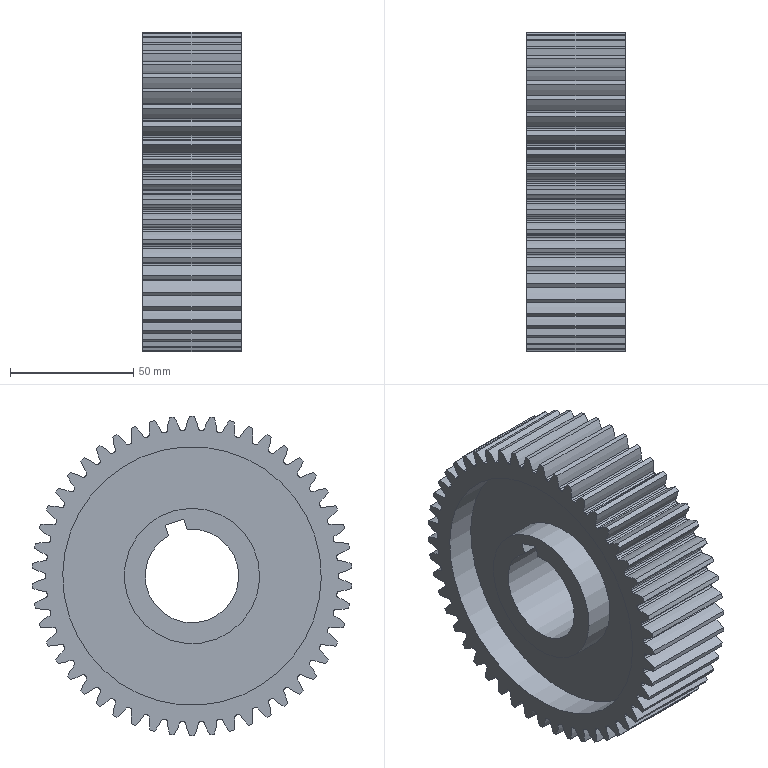Component | NX | CHUANDONGZHOUDACHILUN | 1 solid | 314 faces | volume 288750 mm3 | spline 250 | cylinder 55 | plane 9 | commonest cylinder face diameters 118.63 x50 105 x2 55 x2 38 x1